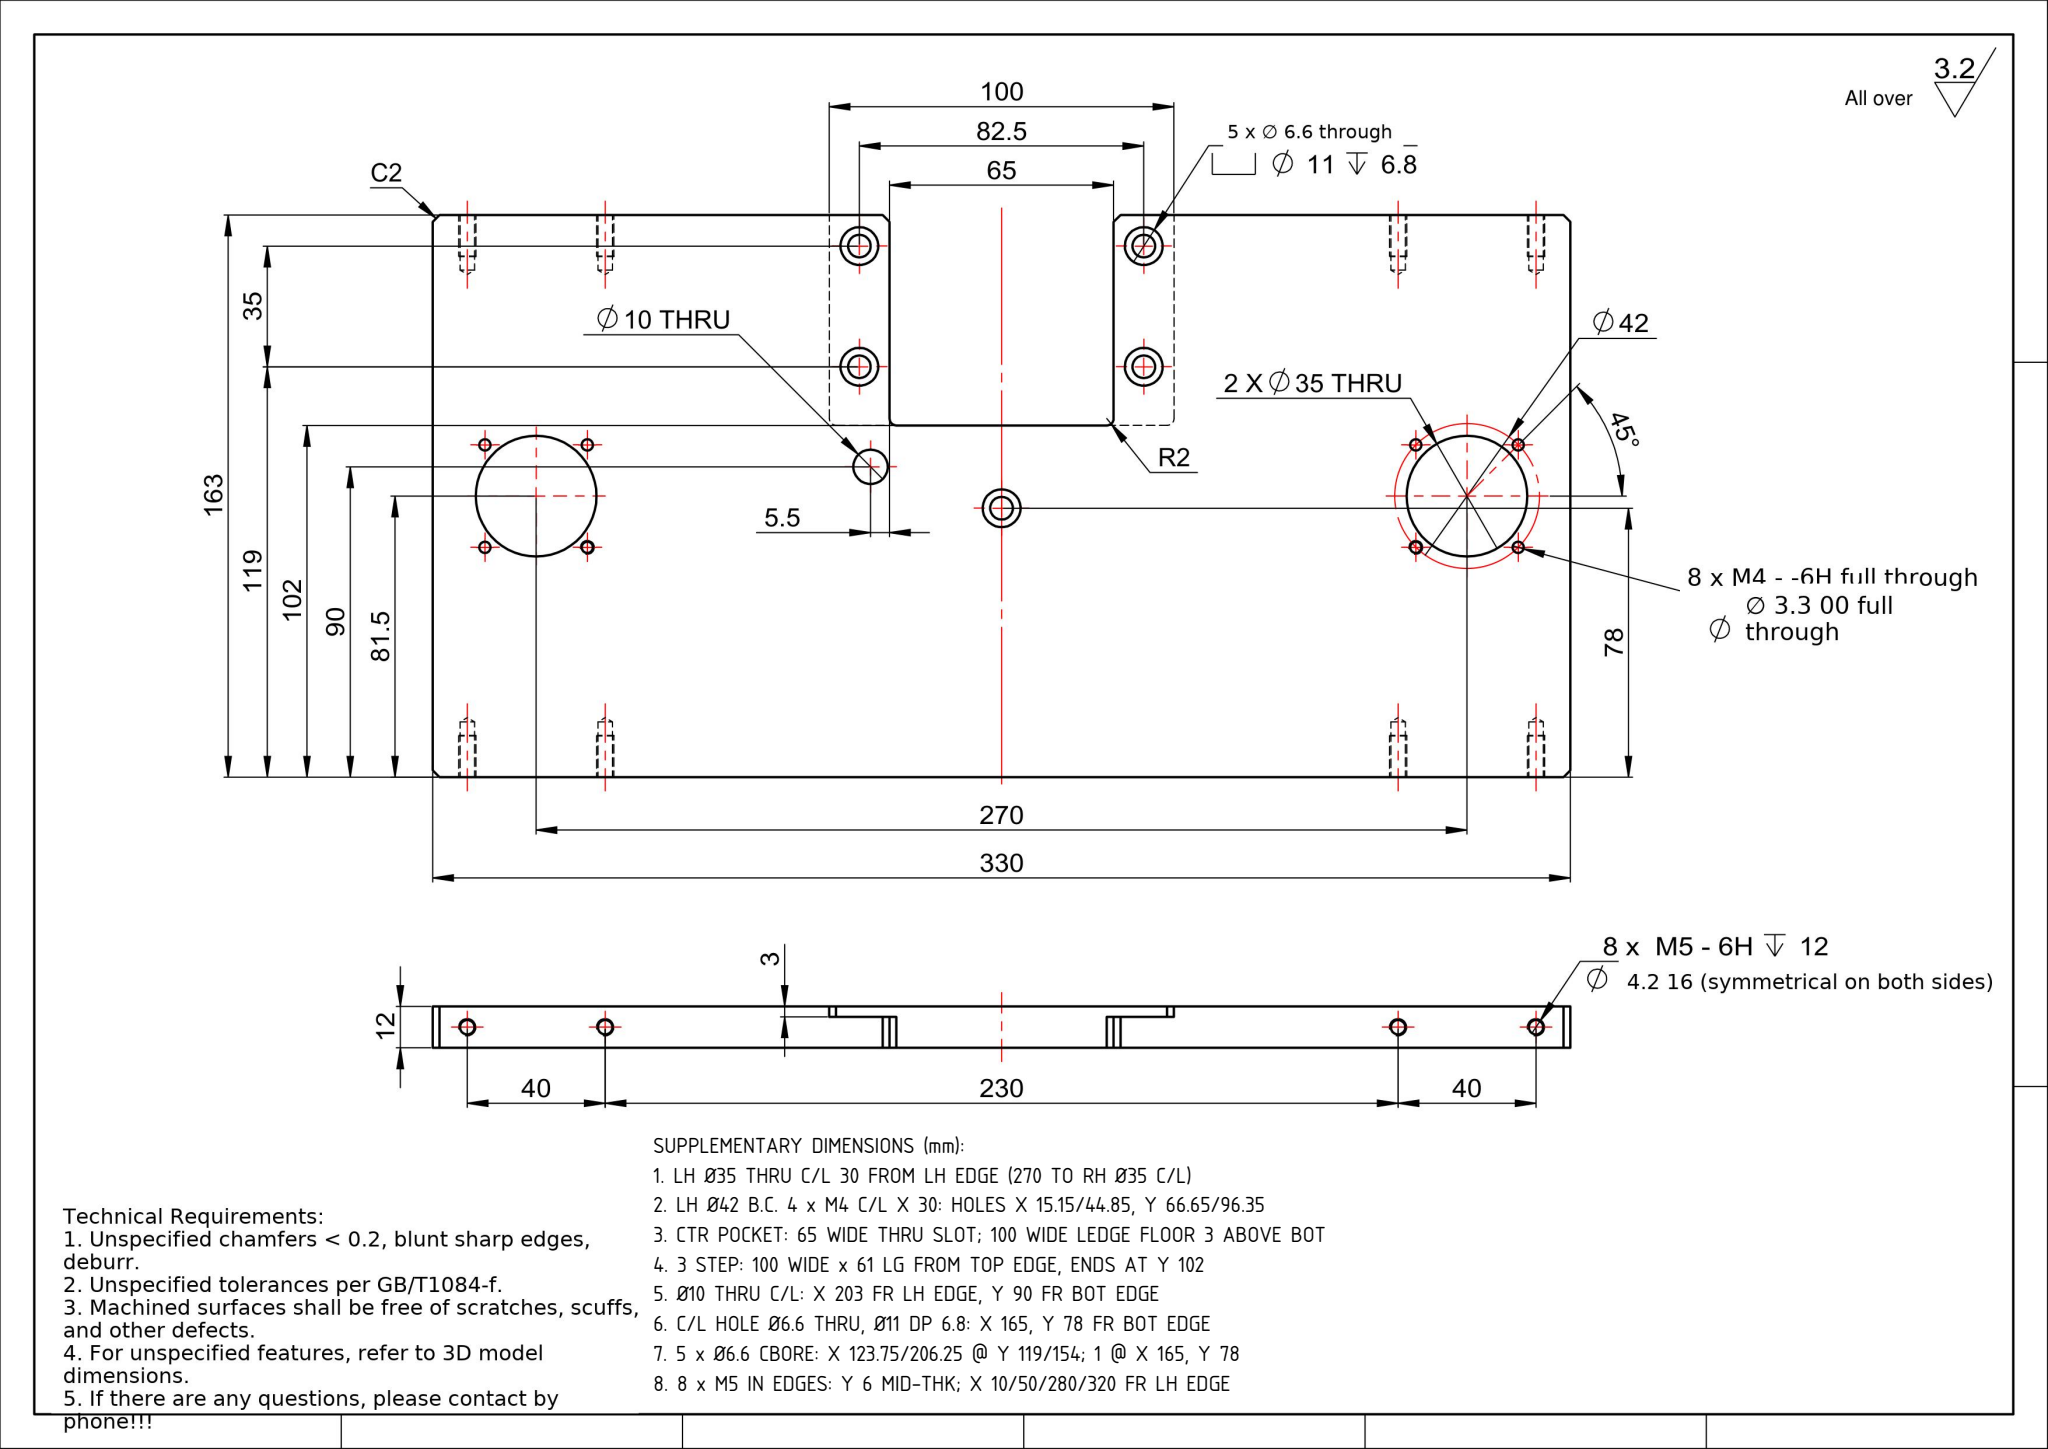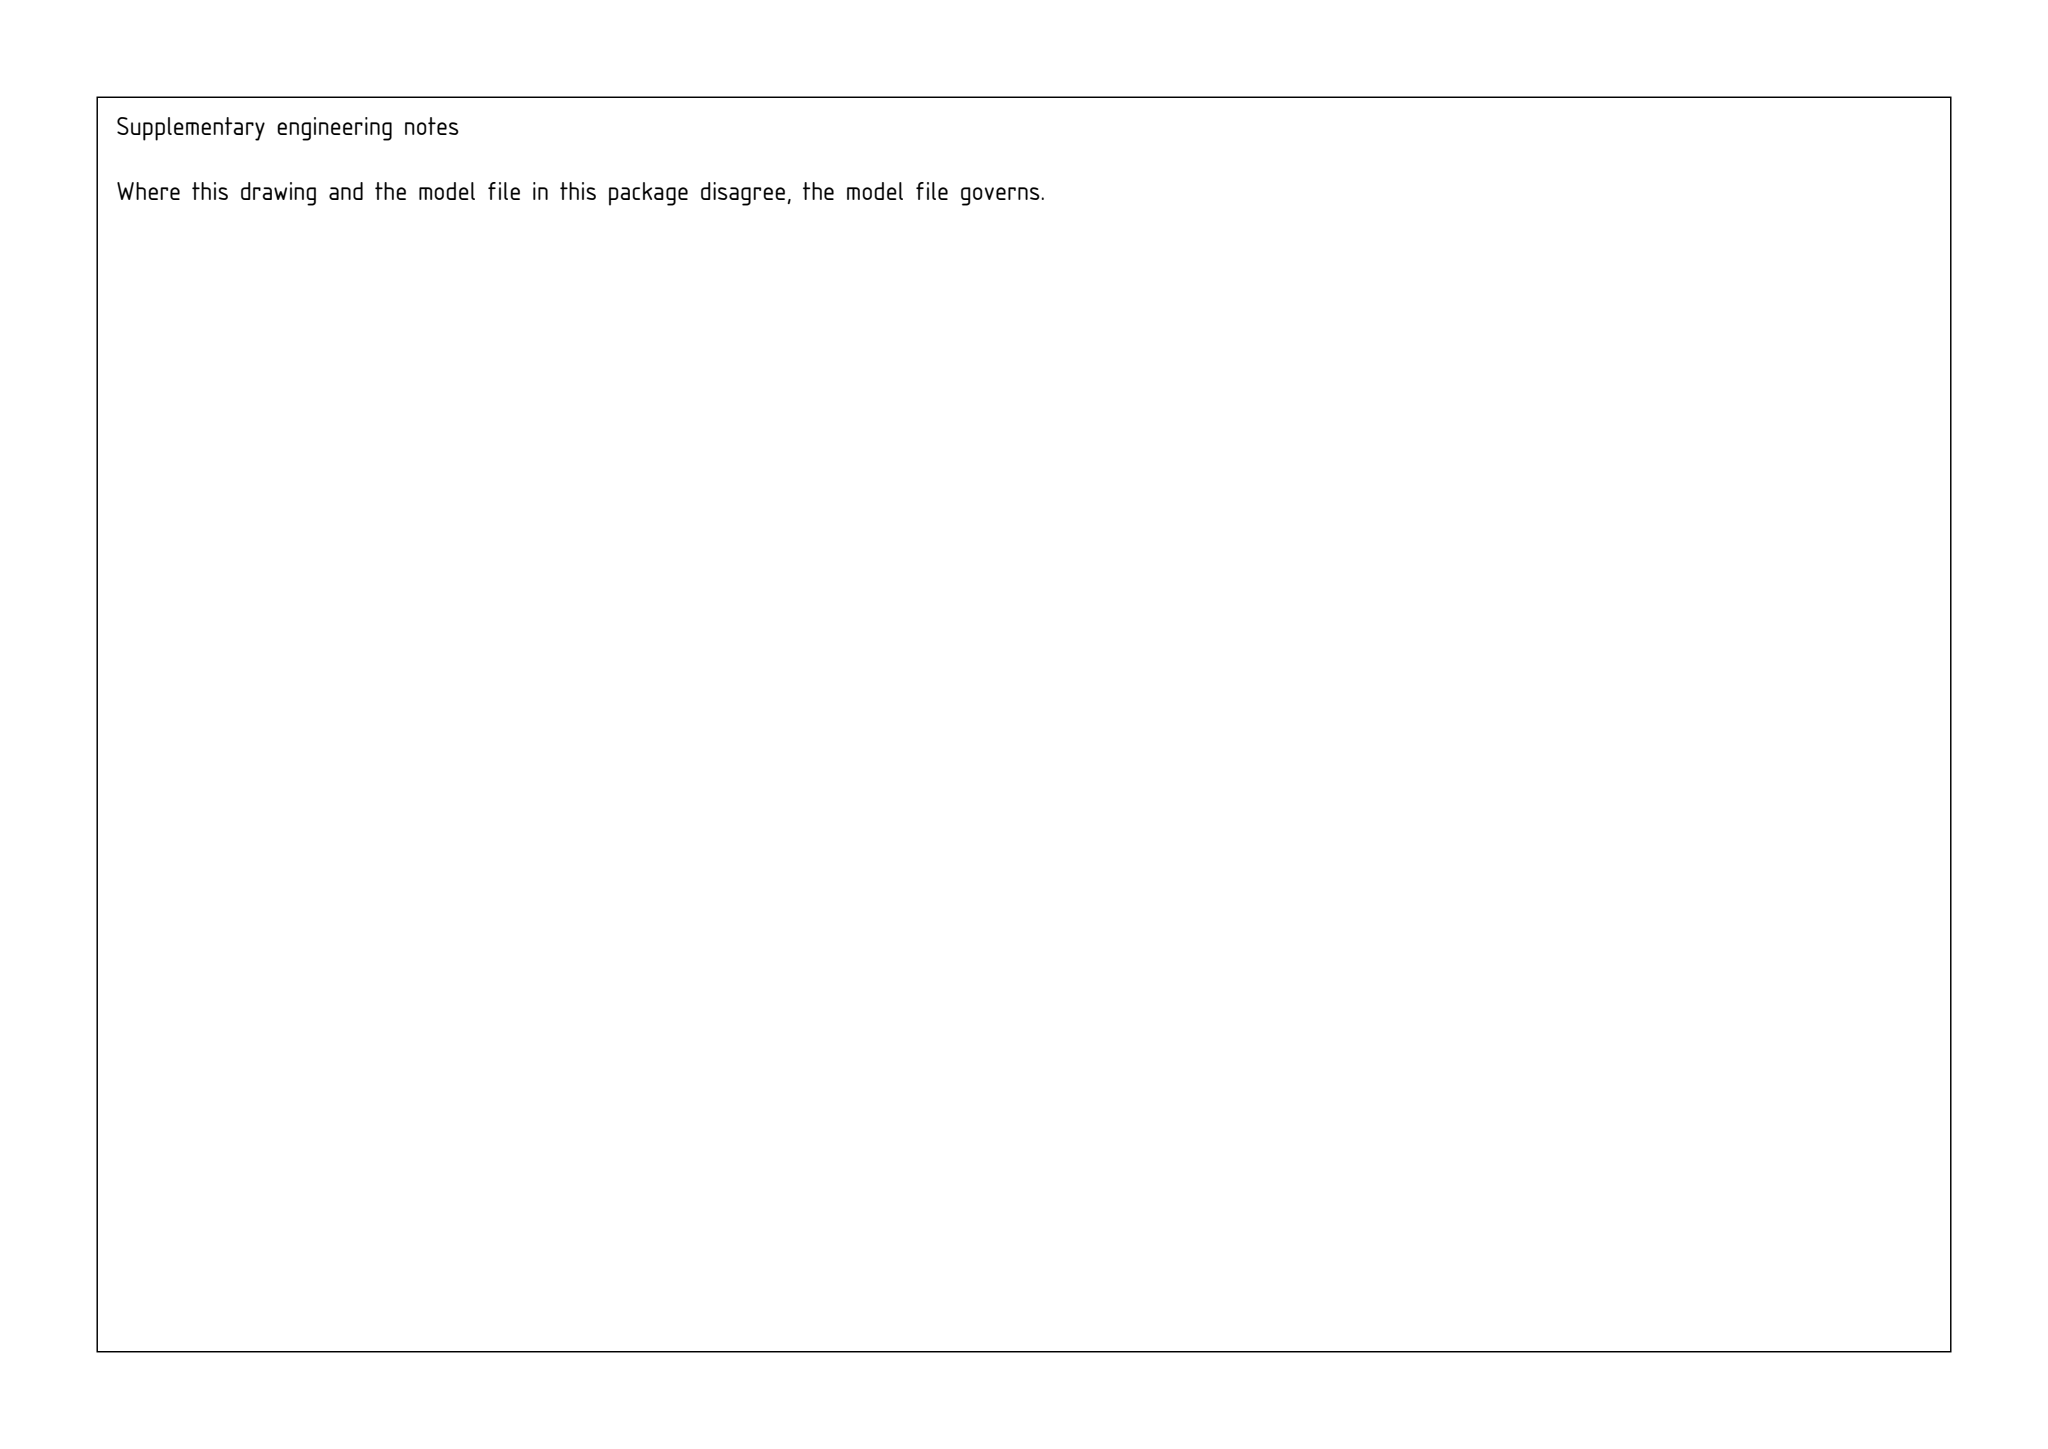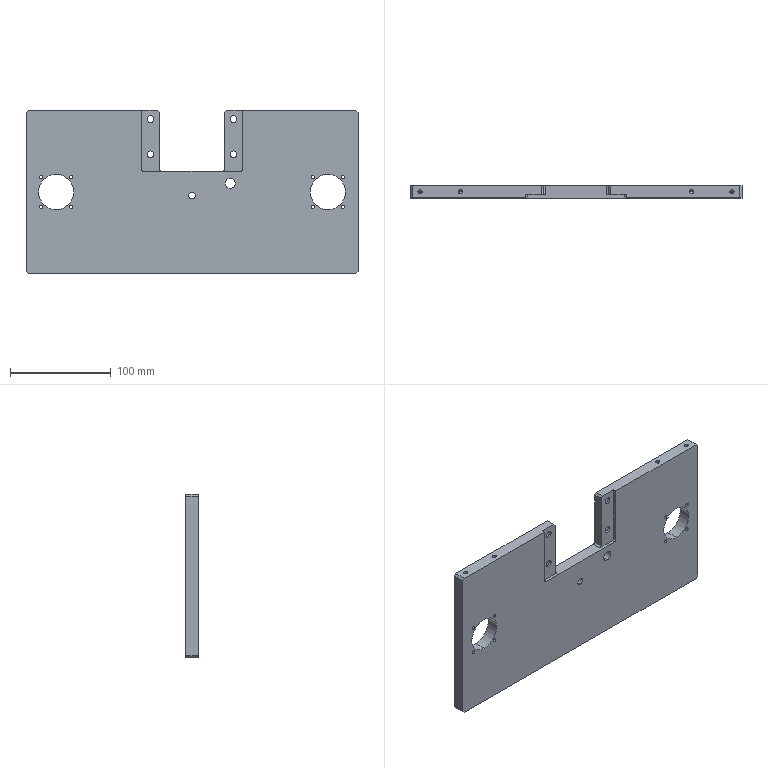Part | SolidWorks | mm | 1 solid | 103 faces | box 330 x 12 x 163 mm | volume 560999 mm3 | cylinder 62 | plane 25 | cone 16 | commonest cylinder face diameters 4.2 x16 3.3 x16 11 x10 6.6 x10 35 x4 4 x4 10 x2
build123d program:
from build123d import *

# Parameters (mm, degrees)
SKETCH1_W                                         = 330
SKETCH1_H                                         = 163
BOSS_EXTRUDE1_DEPTH                               = 6
SKETCH2_W                                         = 65
SKETCH2_H                                         = 65
CUT_EXTRUDE1_DEPTH                                = 185.421
SKETCH3_W                                         = 17.5
SKETCH3_H                                         = 3
CUT_EXTRUDE2_DEPTH                                = 61
SKETCH9_R                                         = 17.5
CUT_EXTRUDE5_DEPTH                                = 185.421
M4_TAPPED_HOLE1_D                                 = 3.3
M5_TAPPED_HOLE1_AT_2_COUNT                        = 2
M5_TAPPED_HOLE1_AT_2_PITCH                        = 40
M5_TAPPED_HOLE1_AT_3_COUNT                        = 2
M5_TAPPED_HOLE1_AT_3_PITCH                        = 230
M5_TAPPED_HOLE1_AT_4_COUNT                        = 2
M5_TAPPED_HOLE1_AT_4_PITCH                        = 270
HOLE_SIZE_ACCORDING_TO_TYPE_1_OF_HEXA_D           = 6.6
HOLE_SIZE_ACCORDING_TO_TYPE_1_OF_HEXA_CBORE_D     = 11
HOLE_SIZE_ACCORDING_TO_TYPE_1_OF_HEXA_CBORE_DEPTH = 6.8
CHAMFER1_SIZE                                     = 2
FILLET1_R                                         = 2
FILLET2_R                                         = 2
CHAMFER2_SIZE                                     = 2
F_10_0_10_DIAMETER_HOLE1_D                        = 10
F_10_0_10_DIAMETER_HOLE1_DEPTH                    = 12
F_10_0_10_DIAMETER_HOLE1_TIP                      = 3.004


with BuildPart() as part:
    # Sketch1 → Boss-Extrude1 (new, symmetric)
    with BuildSketch(Plane(origin=(0, 0, 0), x_dir=(1, 0, 0), z_dir=(0, 1, 0))):
        Rectangle(SKETCH1_W, SKETCH1_H)
    extrude(amount=BOSS_EXTRUDE1_DEPTH, both=True)

    # Sketch2 → Cut-Extrude1 (cut, through all)
    with BuildSketch(Plane(origin=(0, 6, 0), x_dir=(1, 0, 0), z_dir=(0, 1, 0))):
        with Locations((0, -53)):
            Rectangle(SKETCH2_W, SKETCH2_H)
    extrude(amount=-CUT_EXTRUDE1_DEPTH, mode=Mode.SUBTRACT)

    # Sketch3 → Cut-Extrude2 (cut)
    with BuildSketch(Plane.XY.offset(81.5)):
        with Locations((-41.25, -4.5)):
            Rectangle(SKETCH3_W, SKETCH3_H)
        with Locations((41.25, -4.5)):
            Rectangle(SKETCH3_W, SKETCH3_H)
    extrude(amount=-CUT_EXTRUDE2_DEPTH, mode=Mode.SUBTRACT)

    # Sketch9 → Cut-Extrude5 (cut, through all)
    with BuildSketch(Plane(origin=(0, 6, 0), x_dir=(1, 0, 0), z_dir=(0, 1, 0))):
        with Locations(Location((-135, 0, 0), (0, 0, 270))):
            Circle(SKETCH9_R)
    cut_extrude5 = extrude(amount=-CUT_EXTRUDE5_DEPTH, mode=Mode.SUBTRACT)

    # M4 Tapped Hole1 (through all)
    with Locations(Plane(origin=(0, -6, 0), x_dir=(-1, 0, 0), z_dir=(0, -1, 0))):
        with Locations((120.151, 14.849), (120.151, -14.849), (149.849, -14.849), (149.849, 14.849)):
            m4_tapped_hole1 = Hole(M4_TAPPED_HOLE1_D / 2)

    # Sketch13 → M5 Tapped Hole1 (revolve, cut)
    with BuildSketch(Plane(origin=(-115, 0, 81.5), x_dir=(0, -1, 0), z_dir=(1, 0, 0))):
        Polygon((0, 0), (0, 17.262), (2.1, 16), (2.1, 0), align=None)
    m5_tapped_hole1 = revolve(axis=Axis((-115, 0, 87.85), (0, 0, -1)), mode=Mode.SUBTRACT)

    # M5 Tapped Hole1 at 2: M5 Tapped Hole1 ×2
    with Locations(*[(-i * M5_TAPPED_HOLE1_AT_2_PITCH, 0, 0) for i in range(1, M5_TAPPED_HOLE1_AT_2_COUNT)]):
        add(m5_tapped_hole1, mode=Mode.SUBTRACT)

    # M5 Tapped Hole1 at 3: M5 Tapped Hole1 ×2
    with Locations(*[(i * M5_TAPPED_HOLE1_AT_3_PITCH, 0, 0) for i in range(1, M5_TAPPED_HOLE1_AT_3_COUNT)]):
        add(m5_tapped_hole1, mode=Mode.SUBTRACT)

    # M5 Tapped Hole1 at 4: M5 Tapped Hole1 ×2
    with Locations(*[(i * M5_TAPPED_HOLE1_AT_4_PITCH, 0, 0) for i in range(1, M5_TAPPED_HOLE1_AT_4_COUNT)]):
        add(m5_tapped_hole1, mode=Mode.SUBTRACT)

    # Mirror1: Cut-Extrude5, M4 Tapped Hole1 across plane
    add(cut_extrude5.mirror(Plane(origin=(0, 0, 0), x_dir=(0, 0, 1), z_dir=(1, 0, 0))), mode=Mode.SUBTRACT)
    add(m4_tapped_hole1.mirror(Plane(origin=(0, 0, 0), x_dir=(0, 0, 1), z_dir=(1, 0, 0))), mode=Mode.SUBTRACT)

    # Mirror2: M5 Tapped Hole1 across plane
    add(m5_tapped_hole1.mirror(Plane.XY), mode=Mode.SUBTRACT)

    # Mirror2 copy 1 sketch → Mirror2 copy 1 (revolve, cut)
    with BuildSketch(Plane(origin=(-155, 0, -81.5), x_dir=(0, -1, 0), z_dir=(1, 0, 0))):
        Polygon((0, 0), (0, -17.262), (2.1, -16), (2.1, 0), align=None)
    revolve(axis=Axis((-155, 0, -87.85), (0, 0, -1)), mode=Mode.SUBTRACT)

    # Mirror2 copy 2 sketch → Mirror2 copy 2 (revolve, cut)
    with BuildSketch(Plane(origin=(115, 0, -81.5), x_dir=(0, -1, 0), z_dir=(1, 0, 0))):
        Polygon((0, 0), (0, -17.262), (2.1, -16), (2.1, 0), align=None)
    revolve(axis=Axis((115, 0, -87.85), (0, 0, -1)), mode=Mode.SUBTRACT)

    # Mirror2 copy 3 sketch → Mirror2 copy 3 (revolve, cut)
    with BuildSketch(Plane(origin=(155, 0, -81.5), x_dir=(0, -1, 0), z_dir=(1, 0, 0))):
        Polygon((0, 0), (0, -17.262), (2.1, -16), (2.1, 0), align=None)
    revolve(axis=Axis((155, 0, -87.85), (0, 0, -1)), mode=Mode.SUBTRACT)

    # Hole Size _ according to_ Type 1 of Hexa (through all)
    with Locations(Plane(origin=(0, 6, 0), x_dir=(-1, 0, 0), z_dir=(0, 1, 0))):
        with Locations((41.25, 72.5), (41.25, 37.5), (-41.25, 72.5), (-41.25, 37.5), (0, -3.5)):
            CounterBoreHole(HOLE_SIZE_ACCORDING_TO_TYPE_1_OF_HEXA_D / 2, HOLE_SIZE_ACCORDING_TO_TYPE_1_OF_HEXA_CBORE_D / 2, HOLE_SIZE_ACCORDING_TO_TYPE_1_OF_HEXA_CBORE_DEPTH)

    # Chamfer1
    chamfer1_edges = [part.edges().sort_by_distance(p)[0] for p in [
        (32.5, 1.5, 81.5),
        (-32.5, 1.5, 81.5),
    ]]
    chamfer(chamfer1_edges, length=CHAMFER1_SIZE)

    # Fillet1
    fillet1_edges = [part.edges().sort_by_distance(p)[0] for p in [
        (-32.5, 1.5, 20.5),
        (32.5, 1.5, 20.5),
    ]]
    fillet(fillet1_edges, radius=FILLET1_R)

    # Fillet2
    fillet2_edges = [part.edges().sort_by_distance(p)[0] for p in [
        (-50, -4.5, 20.5),
        (50, -4.5, 20.5),
    ]]
    fillet(fillet2_edges, radius=FILLET2_R)

    # Chamfer2
    chamfer2_edges = [part.edges().sort_by_distance(p)[0] for p in [
        (165, 0, 81.5),
        (-165, 0, 81.5),
        (-165, 0, -81.5),
        (165, 0, -81.5),
    ]]
    chamfer(chamfer2_edges, length=CHAMFER2_SIZE)

    # 10.0 _10_ Diameter Hole1
    with Locations(Plane(origin=(0, 6, 0), x_dir=(1, 0, 0), z_dir=(0, 1, 0))):
        with Locations((38, -8.5)):
            Hole(F_10_0_10_DIAMETER_HOLE1_D / 2, depth=F_10_0_10_DIAMETER_HOLE1_DEPTH)
            with Locations((0, 0, -(F_10_0_10_DIAMETER_HOLE1_DEPTH + F_10_0_10_DIAMETER_HOLE1_TIP / 2))):  # 118° drill point
                Cone(0, F_10_0_10_DIAMETER_HOLE1_D / 2, F_10_0_10_DIAMETER_HOLE1_TIP, mode=Mode.SUBTRACT)


solid = part.part